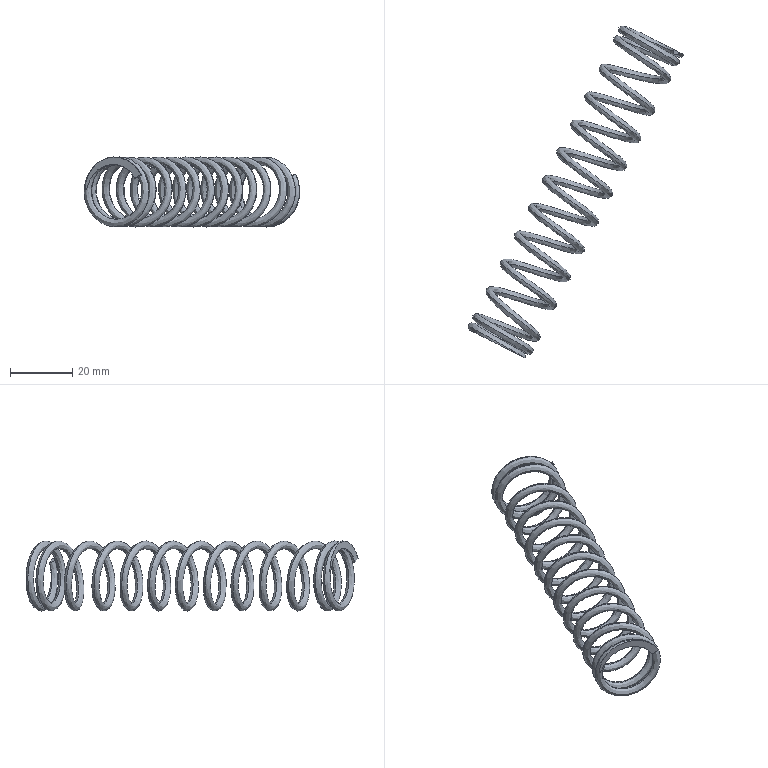Component | SolidWorks | FilmPressingSoilCoveringMechanism2Reverse-2_Spring3-1 | 1 solid | 6 faces | volume 4037 mm3 | plane 4 | spline 2